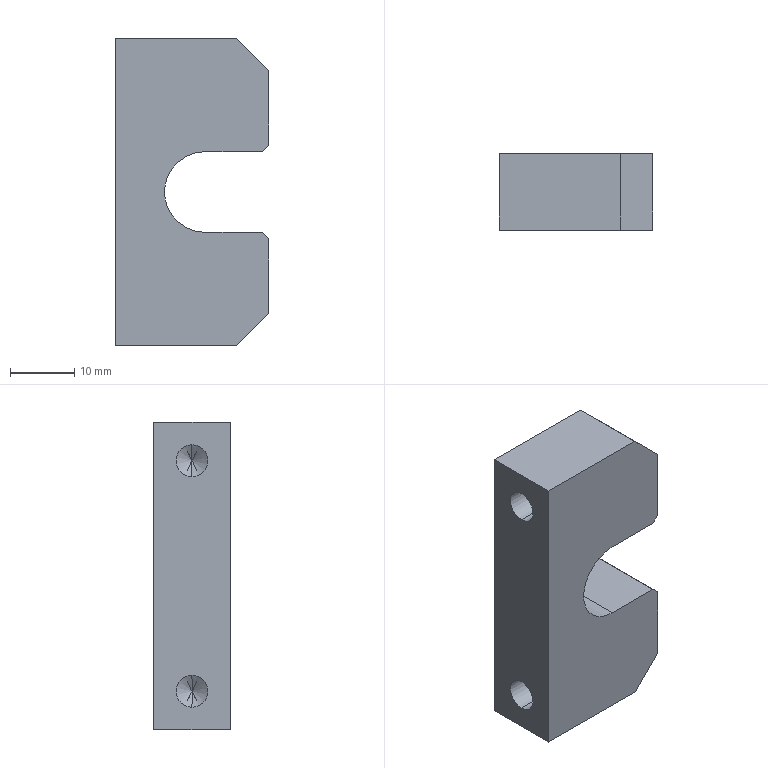Component | SolidWorks | ClampingAssembly-1_A80-1 | 1 solid | 22 faces | box 24 x 12 x 48 mm | volume 10643 mm3 | plane 13 | cylinder 5 | cone 4 | commonest cylinder face diameters 5 x4 12.6 x1 | material S45C
build123d program:
from build123d import *

# Parameters (mm, degrees)
SKETCH1_W             = 48
SKETCH1_H             = 24
BOSS_EXTRUDE1_DEPTH   = 6
M6_TAPPED_HOLE1_D     = 5
M6_TAPPED_HOLE1_DEPTH = 15
M6_TAPPED_HOLE1_TIP   = 1.502
CHAMFER1_SIZE         = 5
CUT_EXTRUDE1_DEPTH    = 30.394
CHAMFER2_SIZE         = 1


with BuildPart() as part:
    # Sketch1 → Boss-Extrude1 (new, symmetric)
    with BuildSketch(Plane(origin=(0, 0, 0), x_dir=(0, 0, -1), z_dir=(1, 0, 0))):
        Rectangle(SKETCH1_W, SKETCH1_H)
    extrude(amount=BOSS_EXTRUDE1_DEPTH, both=True)

    # M6 Tapped Hole1
    with Locations(Plane(origin=(0, -12, 0), x_dir=(-1, 0, 0), z_dir=(0, -1, 0))):
        with Locations((0, -18), (0, 18)):
            Hole(M6_TAPPED_HOLE1_D / 2, depth=M6_TAPPED_HOLE1_DEPTH)
            with Locations((0, 0, -(M6_TAPPED_HOLE1_DEPTH + M6_TAPPED_HOLE1_TIP / 2))):  # 118° drill point
                Cone(0, M6_TAPPED_HOLE1_D / 2, M6_TAPPED_HOLE1_TIP, mode=Mode.SUBTRACT)

    # Chamfer1
    chamfer1_edges = [part.edges().sort_by_distance(p)[0] for p in [
        (0, 12, 24),
        (0, 12, -24),
    ]]
    chamfer(chamfer1_edges, length=CHAMFER1_SIZE)

    # Sketch4 → Cut-Extrude1 (cut, through all)
    with BuildSketch(Plane.ZY.offset(6)):
        with BuildLine():
            Line((6.3, 12), (6.3, 2))
            ThreePointArc((6.3, 2), (0, -4.3), (-6.3, 2))
            Line((-6.3, 2), (-6.3, 12))
            ThreePointArc((-6.3, 12), (0, 18.3), (6.3, 12))
        make_face()
    extrude(amount=-CUT_EXTRUDE1_DEPTH, mode=Mode.SUBTRACT)

    # Chamfer2
    chamfer2_edges = [part.edges().sort_by_distance(p)[0] for p in [
        (0, 12, -6.3),
        (0, 12, 6.3),
    ]]
    chamfer(chamfer2_edges, length=CHAMFER2_SIZE)


solid = part.part

# Placed as in the assembly
solid = solid.moved(Location((7.449, 44.036, -37.5), (0, 0, -90)))
STEP:
#1=COLOUR_RGB('',0.7922,0.8196,0.9333);
#2=FILL_AREA_STYLE_COLOUR('',#1);
#3=FILL_AREA_STYLE('',(#2));
#4=SURFACE_STYLE_FILL_AREA(#3);
#5=SURFACE_SIDE_STYLE('',(#4));
#6=SURFACE_STYLE_USAGE(.BOTH.,#5);
#7=PRESENTATION_STYLE_ASSIGNMENT((#6));
#8=CARTESIAN_POINT('',(0.4114,1.734,-2.283));
#9=VERTEX_POINT('',#8);
#10=CARTESIAN_POINT('',(0.4114,1.734,-2.087));
#11=VERTEX_POINT('',#10);
#12=CARTESIAN_POINT('',(0.4114,1.734,-2.185));
#13=DIRECTION('',(-1.,0.,-0.));
#14=DIRECTION('',(0.,0.,1.));
#15=AXIS2_PLACEMENT_3D('',#12,#13,#14);
#16=CIRCLE('',#15,0.09843);
#17=EDGE_CURVE('',#9,#11,#16,.T.);
#18=ORIENTED_EDGE('',*,*,#17,.F.);
#19=CARTESIAN_POINT('',(-0.1792,1.734,-2.283));
#20=VERTEX_POINT('',#19);
#21=CARTESIAN_POINT('',(-0.1792,1.734,-2.283));
#22=DIRECTION('',(-1.,0.,-0.));
#23=VECTOR('',#22,39.37);
#24=LINE('',#21,#23);
#25=EDGE_CURVE('',#9,#20,#24,.T.);
#26=ORIENTED_EDGE('',*,*,#25,.T.);
#27=CARTESIAN_POINT('',(-0.1792,1.734,-2.087));
#28=VERTEX_POINT('',#27);
#29=CARTESIAN_POINT('',(-0.1792,1.734,-2.185));
#30=DIRECTION('',(-1.,0.,-0.));
#31=DIRECTION('',(0.,0.,1.));
#32=AXIS2_PLACEMENT_3D('',#29,#30,#31);
#33=CIRCLE('',#32,0.09843);
#34=EDGE_CURVE('',#20,#28,#33,.T.);
#35=ORIENTED_EDGE('',*,*,#34,.T.);
#36=CARTESIAN_POINT('',(-0.1792,1.734,-2.087));
#37=DIRECTION('',(-1.,0.,-0.));
#38=VECTOR('',#37,39.37);
#39=LINE('',#36,#38);
#40=EDGE_CURVE('',#11,#28,#39,.T.);
#41=ORIENTED_EDGE('',*,*,#40,.F.);
#42=EDGE_LOOP('',(#18,#26,#35,#41));
#43=FACE_OUTER_BOUND('',#42,.T.);
#44=CARTESIAN_POINT('',(-0.1792,1.734,-2.185));
#45=DIRECTION('',(-1.,0.,-0.));
#46=DIRECTION('',(0.,0.,1.));
#47=AXIS2_PLACEMENT_3D('',#44,#45,#46);
#48=CYLINDRICAL_SURFACE('',#47,0.09843);
#49=ADVANCED_FACE('',(#43),#48,.F.);
#50=CARTESIAN_POINT('',(0.4705,1.734,-2.185));
#51=VERTEX_POINT('',#50);
#52=CARTESIAN_POINT('',(0.4114,1.734,-2.087));
#53=DIRECTION('',(-0.515,0.,0.8572));
#54=VECTOR('',#53,39.37);
#55=LINE('',#52,#54);
#56=EDGE_CURVE('',#51,#11,#55,.T.);
#57=ORIENTED_EDGE('',*,*,#56,.F.);
#58=CARTESIAN_POINT('',(0.4114,1.734,-2.283));
#59=DIRECTION('',(-0.515,0.,-0.8572));
#60=VECTOR('',#59,39.37);
#61=LINE('',#58,#60);
#62=EDGE_CURVE('',#51,#9,#61,.T.);
#63=ORIENTED_EDGE('',*,*,#62,.T.);
#64=ORIENTED_EDGE('',*,*,#17,.T.);
#65=EDGE_LOOP('',(#57,#63,#64));
#66=FACE_OUTER_BOUND('',#65,.T.);
#67=CARTESIAN_POINT('',(0.4114,1.734,-2.185));
#68=DIRECTION('',(-1.,0.,-0.));
#69=DIRECTION('',(0.,0.,1.));
#70=AXIS2_PLACEMENT_3D('',#67,#68,#69);
#71=CONICAL_SURFACE('',#70,0.09843,1.03);
#72=ADVANCED_FACE('',(#66),#71,.F.);
#73=CARTESIAN_POINT('',(0.4114,1.734,-0.8661));
#74=VERTEX_POINT('',#73);
#75=CARTESIAN_POINT('',(0.4114,1.734,-0.6693));
#76=VERTEX_POINT('',#75);
#77=CARTESIAN_POINT('',(0.4114,1.734,-0.7677));
#78=DIRECTION('',(-1.,0.,-0.));
#79=DIRECTION('',(0.,0.,1.));
#80=AXIS2_PLACEMENT_3D('',#77,#78,#79);
#81=CIRCLE('',#80,0.09843);
#82=EDGE_CURVE('',#74,#76,#81,.T.);
#83=ORIENTED_EDGE('',*,*,#82,.F.);
#84=CARTESIAN_POINT('',(-0.1792,1.734,-0.8661));
#85=VERTEX_POINT('',#84);
#86=CARTESIAN_POINT('',(-0.1792,1.734,-0.8661));
#87=DIRECTION('',(-1.,0.,-0.));
#88=VECTOR('',#87,39.37);
#89=LINE('',#86,#88);
#90=EDGE_CURVE('',#74,#85,#89,.T.);
#91=ORIENTED_EDGE('',*,*,#90,.T.);
#92=CARTESIAN_POINT('',(-0.1792,1.734,-0.6693));
#93=VERTEX_POINT('',#92);
#94=CARTESIAN_POINT('',(-0.1792,1.734,-0.7677));
#95=DIRECTION('',(-1.,0.,-0.));
#96=DIRECTION('',(0.,0.,1.));
#97=AXIS2_PLACEMENT_3D('',#94,#95,#96);
#98=CIRCLE('',#97,0.09843);
#99=EDGE_CURVE('',#85,#93,#98,.T.);
#100=ORIENTED_EDGE('',*,*,#99,.T.);
#101=CARTESIAN_POINT('',(-0.1792,1.734,-0.6693));
#102=DIRECTION('',(-1.,0.,-0.));
#103=VECTOR('',#102,39.37);
#104=LINE('',#101,#103);
#105=EDGE_CURVE('',#76,#93,#104,.T.);
#106=ORIENTED_EDGE('',*,*,#105,.F.);
#107=EDGE_LOOP('',(#83,#91,#100,#106));
#108=FACE_OUTER_BOUND('',#107,.T.);
#109=CARTESIAN_POINT('',(-0.1792,1.734,-0.7677));
#110=DIRECTION('',(-1.,0.,-0.));
#111=DIRECTION('',(0.,0.,1.));
#112=AXIS2_PLACEMENT_3D('',#109,#110,#111);
#113=CYLINDRICAL_SURFACE('',#112,0.09843);
#114=ADVANCED_FACE('',(#108),#113,.F.);
#115=CARTESIAN_POINT('',(0.4705,1.734,-0.7677));
#116=VERTEX_POINT('',#115);
#117=CARTESIAN_POINT('',(0.4114,1.734,-0.6693));
#118=DIRECTION('',(-0.515,0.,0.8572));
#119=VECTOR('',#118,39.37);
#120=LINE('',#117,#119);
#121=EDGE_CURVE('',#116,#76,#120,.T.);
#122=ORIENTED_EDGE('',*,*,#121,.F.);
#123=CARTESIAN_POINT('',(0.4114,1.734,-0.8661));
#124=DIRECTION('',(-0.515,0.,-0.8572));
#125=VECTOR('',#124,39.37);
#126=LINE('',#123,#125);
#127=EDGE_CURVE('',#116,#74,#126,.T.);
#128=ORIENTED_EDGE('',*,*,#127,.T.);
#129=ORIENTED_EDGE('',*,*,#82,.T.);
#130=EDGE_LOOP('',(#122,#128,#129));
#131=FACE_OUTER_BOUND('',#130,.T.);
#132=CARTESIAN_POINT('',(0.4114,1.734,-0.7677));
#133=DIRECTION('',(-1.,0.,-0.));
#134=DIRECTION('',(0.,0.,1.));
#135=AXIS2_PLACEMENT_3D('',#132,#133,#134);
#136=CONICAL_SURFACE('',#135,0.09843,1.03);
#137=ADVANCED_FACE('',(#131),#136,.F.);
#138=CARTESIAN_POINT('',(0.7657,1.97,-1.764));
#139=VERTEX_POINT('',#138);
#140=CARTESIAN_POINT('',(0.7657,1.97,-2.224));
#141=VERTEX_POINT('',#140);
#142=CARTESIAN_POINT('',(0.7657,1.97,-2.421));
#143=DIRECTION('',(0.,-0.,-1.));
#144=VECTOR('',#143,39.37);
#145=LINE('',#142,#144);
#146=EDGE_CURVE('',#139,#141,#145,.T.);
#147=ORIENTED_EDGE('',*,*,#146,.F.);
#148=CARTESIAN_POINT('',(0.7657,1.497,-1.764));
#149=VERTEX_POINT('',#148);
#150=CARTESIAN_POINT('',(0.7657,1.97,-1.764));
#151=DIRECTION('',(-0.,-1.,0.));
#152=VECTOR('',#151,39.37);
#153=LINE('',#150,#152);
#154=EDGE_CURVE('',#139,#149,#153,.T.);
#155=ORIENTED_EDGE('',*,*,#154,.T.);
#156=CARTESIAN_POINT('',(0.7657,1.497,-2.224));
#157=VERTEX_POINT('',#156);
#158=CARTESIAN_POINT('',(0.7657,1.497,-2.421));
#159=DIRECTION('',(0.,-0.,-1.));
#160=VECTOR('',#159,39.37);
#161=LINE('',#158,#160);
#162=EDGE_CURVE('',#149,#157,#161,.T.);
#163=ORIENTED_EDGE('',*,*,#162,.T.);
#164=CARTESIAN_POINT('',(0.7657,1.97,-2.224));
#165=DIRECTION('',(0.,1.,-0.));
#166=VECTOR('',#165,39.37);
#167=LINE('',#164,#166);
#168=EDGE_CURVE('',#157,#141,#167,.T.);
#169=ORIENTED_EDGE('',*,*,#168,.T.);
#170=EDGE_LOOP('',(#147,#155,#163,#169));
#171=FACE_OUTER_BOUND('',#170,.T.);
#172=CARTESIAN_POINT('',(0.7657,1.97,-2.421));
#173=DIRECTION('',(-1.,0.,-0.));
#174=DIRECTION('',(-0.,0.,1.));
#175=AXIS2_PLACEMENT_3D('',#172,#173,#174);
#176=PLANE('',#175);
#177=ADVANCED_FACE('',(#171),#176,.F.);
#178=CARTESIAN_POINT('',(-0.1792,1.497,-0.5315));
#179=VERTEX_POINT('',#178);
#180=CARTESIAN_POINT('',(0.5689,1.497,-0.5315));
#181=VERTEX_POINT('',#180);
#182=CARTESIAN_POINT('',(0.7657,1.497,-0.5315));
#183=DIRECTION('',(1.,-0.,-0.));
#184=VECTOR('',#183,39.37);
#185=LINE('',#182,#184);
#186=EDGE_CURVE('',#179,#181,#185,.T.);
#187=ORIENTED_EDGE('',*,*,#186,.T.);
#188=CARTESIAN_POINT('',(0.5689,1.97,-0.5315));
#189=VERTEX_POINT('',#188);
#190=CARTESIAN_POINT('',(0.5689,1.97,-0.5315));
#191=DIRECTION('',(0.,1.,-0.));
#192=VECTOR('',#191,39.37);
#193=LINE('',#190,#192);
#194=EDGE_CURVE('',#181,#189,#193,.T.);
#195=ORIENTED_EDGE('',*,*,#194,.T.);
#196=CARTESIAN_POINT('',(-0.1792,1.97,-0.5315));
#197=VERTEX_POINT('',#196);
#198=CARTESIAN_POINT('',(0.7657,1.97,-0.5315));
#199=DIRECTION('',(1.,-0.,-0.));
#200=VECTOR('',#199,39.37);
#201=LINE('',#198,#200);
#202=EDGE_CURVE('',#197,#189,#201,.T.);
#203=ORIENTED_EDGE('',*,*,#202,.F.);
#204=CARTESIAN_POINT('',(-0.1792,1.97,-0.5315));
#205=DIRECTION('',(-0.,-1.,0.));
#206=VECTOR('',#205,39.37);
#207=LINE('',#204,#206);
#208=EDGE_CURVE('',#197,#179,#207,.T.);
#209=ORIENTED_EDGE('',*,*,#208,.T.);
#210=EDGE_LOOP('',(#187,#195,#203,#209));
#211=FACE_OUTER_BOUND('',#210,.T.);
#212=CARTESIAN_POINT('',(0.7657,1.97,-0.5315));
#213=DIRECTION('',(-0.,-0.,-1.));
#214=DIRECTION('',(-1.,0.,0.));
#215=AXIS2_PLACEMENT_3D('',#212,#213,#214);
#216=PLANE('',#215);
#217=ADVANCED_FACE('',(#211),#216,.F.);
#218=CARTESIAN_POINT('',(0.7657,1.497,-0.7283));
#219=VERTEX_POINT('',#218);
#220=CARTESIAN_POINT('',(0.7657,1.497,-1.189));
#221=VERTEX_POINT('',#220);
#222=CARTESIAN_POINT('',(0.7657,1.497,-2.421));
#223=DIRECTION('',(0.,-0.,-1.));
#224=VECTOR('',#223,39.37);
#225=LINE('',#222,#224);
#226=EDGE_CURVE('',#219,#221,#225,.T.);
#227=ORIENTED_EDGE('',*,*,#226,.T.);
#228=CARTESIAN_POINT('',(0.7657,1.97,-1.189));
#229=VERTEX_POINT('',#228);
#230=CARTESIAN_POINT('',(0.7657,1.97,-1.189));
#231=DIRECTION('',(0.,1.,-0.));
#232=VECTOR('',#231,39.37);
#233=LINE('',#230,#232);
#234=EDGE_CURVE('',#221,#229,#233,.T.);
#235=ORIENTED_EDGE('',*,*,#234,.T.);
#236=CARTESIAN_POINT('',(0.7657,1.97,-0.7283));
#237=VERTEX_POINT('',#236);
#238=CARTESIAN_POINT('',(0.7657,1.97,-2.421));
#239=DIRECTION('',(0.,-0.,-1.));
#240=VECTOR('',#239,39.37);
#241=LINE('',#238,#240);
#242=EDGE_CURVE('',#237,#229,#241,.T.);
#243=ORIENTED_EDGE('',*,*,#242,.F.);
#244=CARTESIAN_POINT('',(0.7657,1.97,-0.7283));
#245=DIRECTION('',(-0.,-1.,0.));
#246=VECTOR('',#245,39.37);
#247=LINE('',#244,#246);
#248=EDGE_CURVE('',#237,#219,#247,.T.);
#249=ORIENTED_EDGE('',*,*,#248,.T.);
#250=EDGE_LOOP('',(#227,#235,#243,#249));
#251=FACE_OUTER_BOUND('',#250,.T.);
#252=CARTESIAN_POINT('',(0.7657,1.97,-2.421));
#253=DIRECTION('',(-1.,0.,-0.));
#254=DIRECTION('',(-0.,0.,1.));
#255=AXIS2_PLACEMENT_3D('',#252,#253,#254);
#256=PLANE('',#255);
#257=ADVANCED_FACE('',(#251),#256,.F.);
#258=CARTESIAN_POINT('',(0.5689,1.97,-2.421));
#259=VERTEX_POINT('',#258);
#260=CARTESIAN_POINT('',(-0.1792,1.97,-2.421));
#261=VERTEX_POINT('',#260);
#262=CARTESIAN_POINT('',(0.7657,1.97,-2.421));
#263=DIRECTION('',(-1.,0.,-0.));
#264=VECTOR('',#263,39.37);
#265=LINE('',#262,#264);
#266=EDGE_CURVE('',#259,#261,#265,.T.);
#267=ORIENTED_EDGE('',*,*,#266,.F.);
#268=CARTESIAN_POINT('',(0.5689,1.497,-2.421));
#269=VERTEX_POINT('',#268);
#270=CARTESIAN_POINT('',(0.5689,1.97,-2.421));
#271=DIRECTION('',(-0.,-1.,0.));
#272=VECTOR('',#271,39.37);
#273=LINE('',#270,#272);
#274=EDGE_CURVE('',#259,#269,#273,.T.);
#275=ORIENTED_EDGE('',*,*,#274,.T.);
#276=CARTESIAN_POINT('',(-0.1792,1.497,-2.421));
#277=VERTEX_POINT('',#276);
#278=CARTESIAN_POINT('',(0.7657,1.497,-2.421));
#279=DIRECTION('',(-1.,0.,-0.));
#280=VECTOR('',#279,39.37);
#281=LINE('',#278,#280);
#282=EDGE_CURVE('',#269,#277,#281,.T.);
#283=ORIENTED_EDGE('',*,*,#282,.T.);
#284=CARTESIAN_POINT('',(-0.1792,1.97,-2.421));
#285=DIRECTION('',(-0.,-1.,0.));
#286=VECTOR('',#285,39.37);
#287=LINE('',#284,#286);
#288=EDGE_CURVE('',#261,#277,#287,.T.);
#289=ORIENTED_EDGE('',*,*,#288,.F.);
#290=EDGE_LOOP('',(#267,#275,#283,#289));
#291=FACE_OUTER_BOUND('',#290,.T.);
#292=CARTESIAN_POINT('',(0.7657,1.97,-2.421));
#293=DIRECTION('',(-0.,0.,1.));
#294=DIRECTION('',(-0.,-1.,0.));
#295=AXIS2_PLACEMENT_3D('',#292,#293,#294);
#296=PLANE('',#295);
#297=ADVANCED_FACE('',(#291),#296,.F.);
#298=CARTESIAN_POINT('',(-0.1792,1.734,-2.185));
#299=DIRECTION('',(-1.,0.,-0.));
#300=DIRECTION('',(0.,0.,1.));
#301=AXIS2_PLACEMENT_3D('',#298,#299,#300);
#302=CIRCLE('',#301,0.09843);
#303=EDGE_CURVE('',#28,#20,#302,.T.);
#304=ORIENTED_EDGE('',*,*,#303,.F.);
#305=ORIENTED_EDGE('',*,*,#34,.F.);
#306=EDGE_LOOP('',(#304,#305));
#307=FACE_BOUND('',#306,.T.);
#308=CARTESIAN_POINT('',(-0.1792,1.734,-0.7677));
#309=DIRECTION('',(-1.,0.,-0.));
#310=DIRECTION('',(0.,0.,1.));
#311=AXIS2_PLACEMENT_3D('',#308,#309,#310);
#312=CIRCLE('',#311,0.09843);
#313=EDGE_CURVE('',#93,#85,#312,.T.);
#314=ORIENTED_EDGE('',*,*,#313,.F.);
#315=ORIENTED_EDGE('',*,*,#99,.F.);
#316=EDGE_LOOP('',(#314,#315));
#317=FACE_BOUND('',#316,.T.);
#318=CARTESIAN_POINT('',(-0.1792,1.497,-2.421));
#319=DIRECTION('',(-0.,0.,1.));
#320=VECTOR('',#319,39.37);
#321=LINE('',#318,#320);
#322=EDGE_CURVE('',#277,#179,#321,.T.);
#323=ORIENTED_EDGE('',*,*,#322,.T.);
#324=ORIENTED_EDGE('',*,*,#208,.F.);
#325=CARTESIAN_POINT('',(-0.1792,1.97,-2.421));
#326=DIRECTION('',(-0.,0.,1.));
#327=VECTOR('',#326,39.37);
#328=LINE('',#325,#327);
#329=EDGE_CURVE('',#261,#197,#328,.T.);
#330=ORIENTED_EDGE('',*,*,#329,.F.);
#331=ORIENTED_EDGE('',*,*,#288,.T.);
#332=EDGE_LOOP('',(#323,#324,#330,#331));
#333=FACE_OUTER_BOUND('',#332,.T.);
#334=CARTESIAN_POINT('',(-0.1792,1.97,-2.421));
#335=DIRECTION('',(1.,-0.,0.));
#336=DIRECTION('',(0.,-0.,-1.));
#337=AXIS2_PLACEMENT_3D('',#334,#335,#336);
#338=PLANE('',#337);
#339=ADVANCED_FACE('',(#307,#317,#333),#338,.F.);
#340=CARTESIAN_POINT('',(0.372,1.97,-1.724));
#341=VERTEX_POINT('',#340);
#342=CARTESIAN_POINT('',(0.7263,1.97,-1.724));
#343=VERTEX_POINT('',#342);
#344=CARTESIAN_POINT('',(0.7657,1.97,-1.724));
#345=DIRECTION('',(1.,-0.,0.));
#346=VECTOR('',#345,39.37);
#347=LINE('',#344,#346);
#348=EDGE_CURVE('',#341,#343,#347,.T.);
#349=ORIENTED_EDGE('',*,*,#348,.T.);
#350=CARTESIAN_POINT('',(0.3858,1.97,-1.384));
#351=DIRECTION('',(0.7071,-0.,-0.7071));
#352=VECTOR('',#351,39.37);
#353=LINE('',#350,#352);
#354=EDGE_CURVE('',#343,#139,#353,.T.);
#355=ORIENTED_EDGE('',*,*,#354,.T.);
#356=ORIENTED_EDGE('',*,*,#146,.T.);
#357=CARTESIAN_POINT('',(0.9035,1.97,-2.087));
#358=DIRECTION('',(-0.7071,-0.,-0.7071));
#359=VECTOR('',#358,39.37);
#360=LINE('',#357,#359);
#361=EDGE_CURVE('',#141,#259,#360,.T.);
#362=ORIENTED_EDGE('',*,*,#361,.T.);
#363=ORIENTED_EDGE('',*,*,#266,.T.);
#364=ORIENTED_EDGE('',*,*,#329,.T.);
#365=ORIENTED_EDGE('',*,*,#202,.T.);
#366=CARTESIAN_POINT('',(0.9035,1.97,-0.8661));
#367=DIRECTION('',(0.7071,-0.,-0.7071));
#368=VECTOR('',#367,39.37);
#369=LINE('',#366,#368);
#370=EDGE_CURVE('',#189,#237,#369,.T.);
#371=ORIENTED_EDGE('',*,*,#370,.T.);
#372=ORIENTED_EDGE('',*,*,#242,.T.);
#373=CARTESIAN_POINT('',(0.7263,1.97,-1.228));
#374=VERTEX_POINT('',#373);
#375=CARTESIAN_POINT('',(0.3858,1.97,-1.569));
#376=DIRECTION('',(-0.7071,-0.,-0.7071));
#377=VECTOR('',#376,39.37);
#378=LINE('',#375,#377);
#379=EDGE_CURVE('',#229,#374,#378,.T.);
#380=ORIENTED_EDGE('',*,*,#379,.T.);
#381=CARTESIAN_POINT('',(0.372,1.97,-1.228));
#382=VERTEX_POINT('',#381);
#383=CARTESIAN_POINT('',(0.7657,1.97,-1.228));
#384=DIRECTION('',(-1.,0.,-0.));
#385=VECTOR('',#384,39.37);
#386=LINE('',#383,#385);
#387=EDGE_CURVE('',#374,#382,#386,.T.);
#388=ORIENTED_EDGE('',*,*,#387,.T.);
#389=CARTESIAN_POINT('',(0.372,1.97,-1.476));
#390=DIRECTION('',(-0.,-1.,0.));
#391=DIRECTION('',(0.,0.,-1.));
#392=AXIS2_PLACEMENT_3D('',#389,#390,#391);
#393=CIRCLE('',#392,0.248);
#394=EDGE_CURVE('',#382,#341,#393,.T.);
#395=ORIENTED_EDGE('',*,*,#394,.T.);
#396=EDGE_LOOP('',(#349,#355,#356,#362,#363,#364,#365,#371,#372,#380,#388,#395));
#397=FACE_OUTER_BOUND('',#396,.T.);
#398=CARTESIAN_POINT('',(0.2933,1.97,-1.476));
#399=DIRECTION('',(0.,1.,-0.));
#400=DIRECTION('',(-0.,0.,1.));
#401=AXIS2_PLACEMENT_3D('',#398,#399,#400);
#402=PLANE('',#401);
#403=ADVANCED_FACE('',(#397),#402,.T.);
#404=ORIENTED_EDGE('',*,*,#162,.F.);
#405=CARTESIAN_POINT('',(0.7263,1.497,-1.724));
#406=VERTEX_POINT('',#405);
#407=CARTESIAN_POINT('',(0.7657,1.497,-1.764));
#408=DIRECTION('',(-0.7071,0.,0.7071));
#409=VECTOR('',#408,39.37);
#410=LINE('',#407,#409);
#411=EDGE_CURVE('',#149,#406,#410,.T.);
#412=ORIENTED_EDGE('',*,*,#411,.T.);
#413=CARTESIAN_POINT('',(0.372,1.497,-1.724));
#414=VERTEX_POINT('',#413);
#415=CARTESIAN_POINT('',(0.7657,1.497,-1.724));
#416=DIRECTION('',(1.,-0.,0.));
#417=VECTOR('',#416,39.37);
#418=LINE('',#415,#417);
#419=EDGE_CURVE('',#414,#406,#418,.T.);
#420=ORIENTED_EDGE('',*,*,#419,.F.);
#421=CARTESIAN_POINT('',(0.372,1.497,-1.228));
#422=VERTEX_POINT('',#421);
#423=CARTESIAN_POINT('',(0.372,1.497,-1.476));
#424=DIRECTION('',(-0.,-1.,0.));
#425=DIRECTION('',(0.,0.,-1.));
#426=AXIS2_PLACEMENT_3D('',#423,#424,#425);
#427=CIRCLE('',#426,0.248);
#428=EDGE_CURVE('',#422,#414,#427,.T.);
#429=ORIENTED_EDGE('',*,*,#428,.F.);
#430=CARTESIAN_POINT('',(0.7263,1.497,-1.228));
#431=VERTEX_POINT('',#430);
#432=CARTESIAN_POINT('',(0.7657,1.497,-1.228));
#433=DIRECTION('',(-1.,0.,-0.));
#434=VECTOR('',#433,39.37);
#435=LINE('',#432,#434);
#436=EDGE_CURVE('',#431,#422,#435,.T.);
#437=ORIENTED_EDGE('',*,*,#436,.F.);
#438=CARTESIAN_POINT('',(0.7263,1.497,-1.228));
#439=DIRECTION('',(0.7071,0.,0.7071));
#440=VECTOR('',#439,39.37);
#441=LINE('',#438,#440);
#442=EDGE_CURVE('',#431,#221,#441,.T.);
#443=ORIENTED_EDGE('',*,*,#442,.T.);
#444=ORIENTED_EDGE('',*,*,#226,.F.);
#445=CARTESIAN_POINT('',(0.7657,1.497,-0.7283));
#446=DIRECTION('',(-0.7071,0.,0.7071));
#447=VECTOR('',#446,39.37);
#448=LINE('',#445,#447);
#449=EDGE_CURVE('',#219,#181,#448,.T.);
#450=ORIENTED_EDGE('',*,*,#449,.T.);
#451=ORIENTED_EDGE('',*,*,#186,.F.);
#452=ORIENTED_EDGE('',*,*,#322,.F.);
#453=ORIENTED_EDGE('',*,*,#282,.F.);
#454=CARTESIAN_POINT('',(0.5689,1.497,-2.421));
#455=DIRECTION('',(0.7071,0.,0.7071));
#456=VECTOR('',#455,39.37);
#457=LINE('',#454,#456);
#458=EDGE_CURVE('',#269,#157,#457,.T.);
#459=ORIENTED_EDGE('',*,*,#458,.T.);
#460=EDGE_LOOP('',(#404,#412,#420,#429,#437,#443,#444,#450,#451,#452,#453,#459));
#461=FACE_OUTER_BOUND('',#460,.T.);
#462=CARTESIAN_POINT('',(0.2933,1.497,-1.476));
#463=DIRECTION('',(0.,1.,-0.));
#464=DIRECTION('',(-0.,0.,1.));
#465=AXIS2_PLACEMENT_3D('',#462,#463,#464);
#466=PLANE('',#465);
#467=ADVANCED_FACE('',(#461),#466,.F.);
#468=ORIENTED_EDGE('',*,*,#127,.F.);
#469=ORIENTED_EDGE('',*,*,#121,.T.);
#470=CARTESIAN_POINT('',(0.4114,1.734,-0.7677));
#471=DIRECTION('',(-1.,0.,-0.));
#472=DIRECTION('',(0.,0.,1.));
#473=AXIS2_PLACEMENT_3D('',#470,#471,#472);
#474=CIRCLE('',#473,0.09843);
#475=EDGE_CURVE('',#76,#74,#474,.T.);
#476=ORIENTED_EDGE('',*,*,#475,.T.);
#477=EDGE_LOOP('',(#468,#469,#476));
#478=FACE_OUTER_BOUND('',#477,.T.);
#479=CARTESIAN_POINT('',(0.4114,1.734,-0.7677));
#480=DIRECTION('',(-1.,0.,-0.));
#481=DIRECTION('',(0.,0.,1.));
#482=AXIS2_PLACEMENT_3D('',#479,#480,#481);
#483=CONICAL_SURFACE('',#482,0.09843,1.03);
#484=ADVANCED_FACE('',(#478),#483,.F.);
#485=ORIENTED_EDGE('',*,*,#90,.F.);
#486=ORIENTED_EDGE('',*,*,#475,.F.);
#487=ORIENTED_EDGE('',*,*,#105,.T.);
#488=ORIENTED_EDGE('',*,*,#313,.T.);
#489=EDGE_LOOP('',(#485,#486,#487,#488));
#490=FACE_OUTER_BOUND('',#489,.T.);
#491=CARTESIAN_POINT('',(-0.1792,1.734,-0.7677));
#492=DIRECTION('',(-1.,0.,-0.));
#493=DIRECTION('',(0.,0.,1.));
#494=AXIS2_PLACEMENT_3D('',#491,#492,#493);
#495=CYLINDRICAL_SURFACE('',#494,0.09843);
#496=ADVANCED_FACE('',(#490),#495,.F.);
#497=ORIENTED_EDGE('',*,*,#62,.F.);
#498=ORIENTED_EDGE('',*,*,#56,.T.);
#499=CARTESIAN_POINT('',(0.4114,1.734,-2.185));
#500=DIRECTION('',(-1.,0.,-0.));
#501=DIRECTION('',(0.,0.,1.));
#502=AXIS2_PLACEMENT_3D('',#499,#500,#501);
#503=CIRCLE('',#502,0.09843);
#504=EDGE_CURVE('',#11,#9,#503,.T.);
#505=ORIENTED_EDGE('',*,*,#504,.T.);
#506=EDGE_LOOP('',(#497,#498,#505));
#507=FACE_OUTER_BOUND('',#506,.T.);
#508=CARTESIAN_POINT('',(0.4114,1.734,-2.185));
#509=DIRECTION('',(-1.,0.,-0.));
#510=DIRECTION('',(0.,0.,1.));
#511=AXIS2_PLACEMENT_3D('',#508,#509,#510);
#512=CONICAL_SURFACE('',#511,0.09843,1.03);
#513=ADVANCED_FACE('',(#507),#512,.F.);
#514=ORIENTED_EDGE('',*,*,#25,.F.);
#515=ORIENTED_EDGE('',*,*,#504,.F.);
#516=ORIENTED_EDGE('',*,*,#40,.T.);
#517=ORIENTED_EDGE('',*,*,#303,.T.);
#518=EDGE_LOOP('',(#514,#515,#516,#517));
#519=FACE_OUTER_BOUND('',#518,.T.);
#520=CARTESIAN_POINT('',(-0.1792,1.734,-2.185));
#521=DIRECTION('',(-1.,0.,-0.));
#522=DIRECTION('',(0.,0.,1.));
#523=AXIS2_PLACEMENT_3D('',#520,#521,#522);
#524=CYLINDRICAL_SURFACE('',#523,0.09843);
#525=ADVANCED_FACE('',(#519),#524,.F.);
#526=ORIENTED_EDGE('',*,*,#361,.F.);
#527=ORIENTED_EDGE('',*,*,#168,.F.);
#528=ORIENTED_EDGE('',*,*,#458,.F.);
#529=ORIENTED_EDGE('',*,*,#274,.F.);
#530=EDGE_LOOP('',(#526,#527,#528,#529));
#531=FACE_OUTER_BOUND('',#530,.T.);
#532=CARTESIAN_POINT('',(0.5689,1.97,-2.421));
#533=DIRECTION('',(-0.7071,0.,0.7071));
#534=DIRECTION('',(-0.,-1.,0.));
#535=AXIS2_PLACEMENT_3D('',#532,#533,#534);
#536=PLANE('',#535);
#537=ADVANCED_FACE('',(#531),#536,.F.);
#538=ORIENTED_EDGE('',*,*,#370,.F.);
#539=ORIENTED_EDGE('',*,*,#194,.F.);
#540=ORIENTED_EDGE('',*,*,#449,.F.);
#541=ORIENTED_EDGE('',*,*,#248,.F.);
#542=EDGE_LOOP('',(#538,#539,#540,#541));
#543=FACE_OUTER_BOUND('',#542,.T.);
#544=CARTESIAN_POINT('',(0.7657,1.97,-0.7283));
#545=DIRECTION('',(-0.7071,-0.,-0.7071));
#546=DIRECTION('',(-0.,-1.,0.));
#547=AXIS2_PLACEMENT_3D('',#544,#545,#546);
#548=PLANE('',#547);
#549=ADVANCED_FACE('',(#543),#548,.F.);
#550=ORIENTED_EDGE('',*,*,#419,.T.);
#551=CARTESIAN_POINT('',(0.7263,1.97,-1.724));
#552=DIRECTION('',(0.,1.,-0.));
#553=VECTOR('',#552,39.37);
#554=LINE('',#551,#553);
#555=EDGE_CURVE('',#406,#343,#554,.T.);
#556=ORIENTED_EDGE('',*,*,#555,.T.);
#557=ORIENTED_EDGE('',*,*,#348,.F.);
#558=CARTESIAN_POINT('',(0.372,1.97,-1.724));
#559=DIRECTION('',(-0.,-1.,0.));
#560=VECTOR('',#559,39.37);
#561=LINE('',#558,#560);
#562=EDGE_CURVE('',#341,#414,#561,.T.);
#563=ORIENTED_EDGE('',*,*,#562,.T.);
#564=EDGE_LOOP('',(#550,#556,#557,#563));
#565=FACE_OUTER_BOUND('',#564,.T.);
#566=CARTESIAN_POINT('',(0.7657,1.97,-1.724));
#567=DIRECTION('',(0.,-0.,-1.));
#568=DIRECTION('',(-1.,0.,-0.));
#569=AXIS2_PLACEMENT_3D('',#566,#567,#568);
#570=PLANE('',#569);
#571=ADVANCED_FACE('',(#565),#570,.F.);
#572=ORIENTED_EDGE('',*,*,#428,.T.);
#573=ORIENTED_EDGE('',*,*,#562,.F.);
#574=ORIENTED_EDGE('',*,*,#394,.F.);
#575=CARTESIAN_POINT('',(0.372,1.97,-1.228));
#576=DIRECTION('',(-0.,-1.,0.));
#577=VECTOR('',#576,39.37);
#578=LINE('',#575,#577);
#579=EDGE_CURVE('',#382,#422,#578,.T.);
#580=ORIENTED_EDGE('',*,*,#579,.T.);
#581=EDGE_LOOP('',(#572,#573,#574,#580));
#582=FACE_OUTER_BOUND('',#581,.T.);
#583=CARTESIAN_POINT('',(0.372,1.97,-1.476));
#584=DIRECTION('',(-0.,-1.,0.));
#585=DIRECTION('',(0.,0.,-1.));
#586=AXIS2_PLACEMENT_3D('',#583,#584,#585);
#587=CYLINDRICAL_SURFACE('',#586,0.248);
#588=ADVANCED_FACE('',(#582),#587,.F.);
#589=ORIENTED_EDGE('',*,*,#387,.F.);
#590=CARTESIAN_POINT('',(0.7263,1.97,-1.228));
#591=DIRECTION('',(-0.,-1.,0.));
#592=VECTOR('',#591,39.37);
#593=LINE('',#590,#592);
#594=EDGE_CURVE('',#374,#431,#593,.T.);
#595=ORIENTED_EDGE('',*,*,#594,.T.);
#596=ORIENTED_EDGE('',*,*,#436,.T.);
#597=ORIENTED_EDGE('',*,*,#579,.F.);
#598=EDGE_LOOP('',(#589,#595,#596,#597));
#599=FACE_OUTER_BOUND('',#598,.T.);
#600=CARTESIAN_POINT('',(0.7657,1.97,-1.228));
#601=DIRECTION('',(-0.,0.,1.));
#602=DIRECTION('',(1.,-0.,0.));
#603=AXIS2_PLACEMENT_3D('',#600,#601,#602);
#604=PLANE('',#603);
#605=ADVANCED_FACE('',(#599),#604,.F.);
#606=ORIENTED_EDGE('',*,*,#354,.F.);
#607=ORIENTED_EDGE('',*,*,#555,.F.);
#608=ORIENTED_EDGE('',*,*,#411,.F.);
#609=ORIENTED_EDGE('',*,*,#154,.F.);
#610=EDGE_LOOP('',(#606,#607,#608,#609));
#611=FACE_OUTER_BOUND('',#610,.T.);
#612=CARTESIAN_POINT('',(0.7657,1.97,-1.764));
#613=DIRECTION('',(-0.7071,-0.,-0.7071));
#614=DIRECTION('',(-0.,-1.,0.));
#615=AXIS2_PLACEMENT_3D('',#612,#613,#614);
#616=PLANE('',#615);
#617=ADVANCED_FACE('',(#611),#616,.F.);
#618=ORIENTED_EDGE('',*,*,#379,.F.);
#619=ORIENTED_EDGE('',*,*,#234,.F.);
#620=ORIENTED_EDGE('',*,*,#442,.F.);
#621=ORIENTED_EDGE('',*,*,#594,.F.);
#622=EDGE_LOOP('',(#618,#619,#620,#621));
#623=FACE_OUTER_BOUND('',#622,.T.);
#624=CARTESIAN_POINT('',(0.7263,1.97,-1.228));
#625=DIRECTION('',(-0.7071,0.,0.7071));
#626=DIRECTION('',(-0.,-1.,0.));
#627=AXIS2_PLACEMENT_3D('',#624,#625,#626);
#628=PLANE('',#627);
#629=ADVANCED_FACE('',(#623),#628,.F.);
#630=CLOSED_SHELL('',(#49,#72,#114,#137,#177,#217,#257,#297,#339,#403,#467,#484,#496,#513,#525,#537,#549,#571,#588,#605,#617,#629));
#631=MANIFOLD_SOLID_BREP('',#630);
#632=STYLED_ITEM('',(#7),#631);
#633=PRESENTATION_LAYER_ASSIGNMENT('','',(#632));
#634=(LENGTH_UNIT()NAMED_UNIT(*)SI_UNIT($,.METRE.));
#635=LENGTH_MEASURE_WITH_UNIT(LENGTH_MEASURE(0.0254),#634);
#636=DIMENSIONAL_EXPONENTS(1.,0.,0.,0.,0.,0.,0.);
#637=(CONVERSION_BASED_UNIT('',#635)LENGTH_UNIT()NAMED_UNIT(#636));
#638=UNCERTAINTY_MEASURE_WITH_UNIT(LENGTH_MEASURE(0.00001),#637,'','');
#639=(NAMED_UNIT(*)PLANE_ANGLE_UNIT()SI_UNIT($,.RADIAN.));
#640=(NAMED_UNIT(*)SI_UNIT($,.STERADIAN.)SOLID_ANGLE_UNIT());
#641=(GEOMETRIC_REPRESENTATION_CONTEXT(3)GLOBAL_UNCERTAINTY_ASSIGNED_CONTEXT((#638))GLOBAL_UNIT_ASSIGNED_CONTEXT((#637,#639,#640))REPRESENTATION_CONTEXT('',''));
#642=MECHANICAL_DESIGN_GEOMETRIC_PRESENTATION_REPRESENTATION('',(#632),#641);
#643=CARTESIAN_POINT('',(0.,0.,0.));
#644=DIRECTION('',(0.,0.,1.));
#645=DIRECTION('',(1.,0.,0.));
#646=AXIS2_PLACEMENT_3D('',#643,#644,#645);
#647=(LENGTH_UNIT()NAMED_UNIT(*)SI_UNIT($,.METRE.));
#648=LENGTH_MEASURE_WITH_UNIT(LENGTH_MEASURE(0.0254),#647);
#649=DIMENSIONAL_EXPONENTS(1.,0.,0.,0.,0.,0.,0.);
#650=(CONVERSION_BASED_UNIT('',#648)LENGTH_UNIT()NAMED_UNIT(#649));
#651=UNCERTAINTY_MEASURE_WITH_UNIT(LENGTH_MEASURE(0.00001),#650,'','');
#652=(NAMED_UNIT(*)PLANE_ANGLE_UNIT()SI_UNIT($,.RADIAN.));
#653=(NAMED_UNIT(*)SI_UNIT($,.STERADIAN.)SOLID_ANGLE_UNIT());
#654=(GEOMETRIC_REPRESENTATION_CONTEXT(3)GLOBAL_UNCERTAINTY_ASSIGNED_CONTEXT((#651))GLOBAL_UNIT_ASSIGNED_CONTEXT((#650,#652,#653))REPRESENTATION_CONTEXT('',''));
#655=ADVANCED_BREP_SHAPE_REPRESENTATION('',(#631,#646),#654);